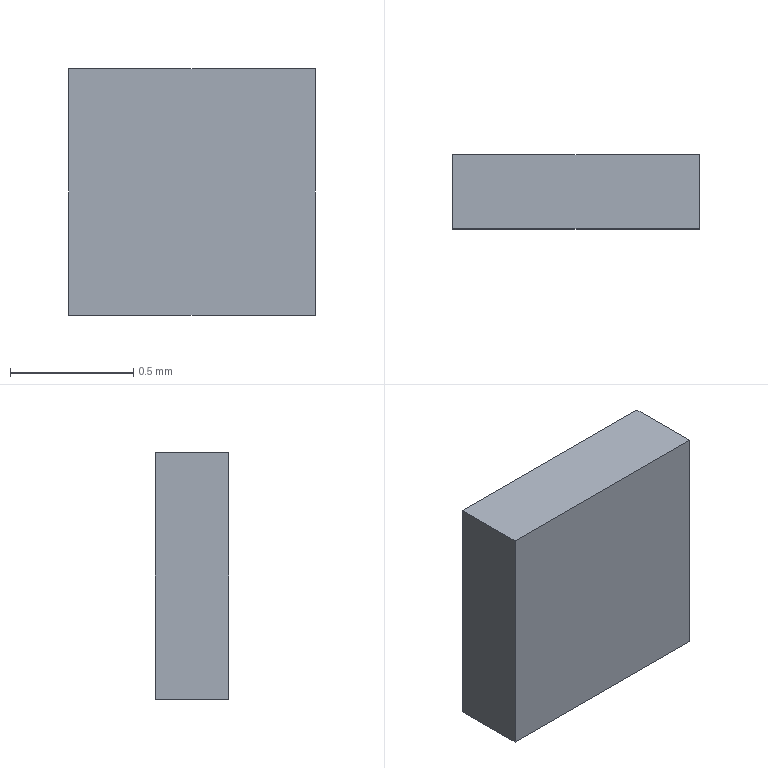Component | NX | SENSOR_21 | 1 solid | 6 faces | box 1 x 0.3 x 1 mm | volume 0 mm3 | plane 6
STEP:
#1=CARTESIAN_POINT('',(0.,0.,0.));
#2=DIRECTION('',(0.,0.,1.));
#3=DIRECTION('',(1.,0.,0.));
#4=AXIS2_PLACEMENT_3D('',#1,#2,#3);
#5=CARTESIAN_POINT('',(-590.087,100.903,1.));
#6=VERTEX_POINT('',#5);
#7=CARTESIAN_POINT('',(-591.087,100.903,1.));
#8=VERTEX_POINT('',#7);
#9=CARTESIAN_POINT('',(-590.587,100.903,1.));
#10=DIRECTION('',(-1.,0.,0.));
#11=VECTOR('',#10,1.);
#12=LINE('',#9,#11);
#13=CARTESIAN_POINT('',(-590.587,101.053,1.));
#14=DIRECTION('',(0.,0.,1.));
#15=DIRECTION('',(1.,0.,0.));
#16=AXIS2_PLACEMENT_3D('',#13,#14,#15);
#17=PLANE('',#16);
#18=CARTESIAN_POINT('',(0.,-0.15));
#19=DIRECTION('',(-1.,0.));
#20=VECTOR('',#19,1.);
#21=LINE('',#18,#20);
#22=(GEOMETRIC_REPRESENTATION_CONTEXT(2)PARAMETRIC_REPRESENTATION_CONTEXT()REPRESENTATION_CONTEXT('',''));
#23=DEFINITIONAL_REPRESENTATION('',(#21),#22);
#24=PCURVE('',#17,#23);
#25=CARTESIAN_POINT('',(-590.587,100.903,0.));
#26=DIRECTION('',(0.,-1.,0.));
#27=DIRECTION('',(0.,0.,-1.));
#28=AXIS2_PLACEMENT_3D('',#25,#26,#27);
#29=PLANE('',#28);
#30=CARTESIAN_POINT('',(-1.,0.));
#31=DIRECTION('',(0.,-1.));
#32=VECTOR('',#31,1.);
#33=LINE('',#30,#32);
#34=(GEOMETRIC_REPRESENTATION_CONTEXT(2)PARAMETRIC_REPRESENTATION_CONTEXT()REPRESENTATION_CONTEXT('',''));
#35=DEFINITIONAL_REPRESENTATION('',(#33),#34);
#36=PCURVE('',#29,#35);
#37=SURFACE_CURVE('',#12,(#24,#36),.PCURVE_S1.);
#38=EDGE_CURVE('',#6,#8,#37,.T.);
#39=ORIENTED_EDGE('',*,*,#38,.F.);
#40=CARTESIAN_POINT('',(-590.087,101.203,1.));
#41=VERTEX_POINT('',#40);
#42=CARTESIAN_POINT('',(-590.087,101.053,1.));
#43=DIRECTION('',(0.,-1.,0.));
#44=VECTOR('',#43,1.);
#45=LINE('',#42,#44);
#46=CARTESIAN_POINT('',(0.5,0.));
#47=DIRECTION('',(0.,-1.));
#48=VECTOR('',#47,1.);
#49=LINE('',#46,#48);
#50=(GEOMETRIC_REPRESENTATION_CONTEXT(2)PARAMETRIC_REPRESENTATION_CONTEXT()REPRESENTATION_CONTEXT('',''));
#51=DEFINITIONAL_REPRESENTATION('',(#49),#50);
#52=PCURVE('',#17,#51);
#53=CARTESIAN_POINT('',(-590.087,101.053,0.));
#54=DIRECTION('',(1.,0.,0.));
#55=DIRECTION('',(0.,0.,-1.));
#56=AXIS2_PLACEMENT_3D('',#53,#54,#55);
#57=PLANE('',#56);
#58=CARTESIAN_POINT('',(-1.,0.));
#59=DIRECTION('',(0.,-1.));
#60=VECTOR('',#59,1.);
#61=LINE('',#58,#60);
#62=(GEOMETRIC_REPRESENTATION_CONTEXT(2)PARAMETRIC_REPRESENTATION_CONTEXT()REPRESENTATION_CONTEXT('',''));
#63=DEFINITIONAL_REPRESENTATION('',(#61),#62);
#64=PCURVE('',#57,#63);
#65=SURFACE_CURVE('',#45,(#52,#64),.PCURVE_S1.);
#66=EDGE_CURVE('',#41,#6,#65,.T.);
#67=ORIENTED_EDGE('',*,*,#66,.F.);
#68=CARTESIAN_POINT('',(-591.087,101.203,1.));
#69=VERTEX_POINT('',#68);
#70=CARTESIAN_POINT('',(-590.587,101.203,1.));
#71=DIRECTION('',(1.,0.,0.));
#72=VECTOR('',#71,1.);
#73=LINE('',#70,#72);
#74=CARTESIAN_POINT('',(0.,0.15));
#75=DIRECTION('',(1.,0.));
#76=VECTOR('',#75,1.);
#77=LINE('',#74,#76);
#78=(GEOMETRIC_REPRESENTATION_CONTEXT(2)PARAMETRIC_REPRESENTATION_CONTEXT()REPRESENTATION_CONTEXT('',''));
#79=DEFINITIONAL_REPRESENTATION('',(#77),#78);
#80=PCURVE('',#17,#79);
#81=CARTESIAN_POINT('',(-590.587,101.203,0.));
#82=DIRECTION('',(0.,1.,0.));
#83=DIRECTION('',(0.,0.,1.));
#84=AXIS2_PLACEMENT_3D('',#81,#82,#83);
#85=PLANE('',#84);
#86=CARTESIAN_POINT('',(1.,0.));
#87=DIRECTION('',(0.,1.));
#88=VECTOR('',#87,1.);
#89=LINE('',#86,#88);
#90=(GEOMETRIC_REPRESENTATION_CONTEXT(2)PARAMETRIC_REPRESENTATION_CONTEXT()REPRESENTATION_CONTEXT('',''));
#91=DEFINITIONAL_REPRESENTATION('',(#89),#90);
#92=PCURVE('',#85,#91);
#93=SURFACE_CURVE('',#73,(#80,#92),.PCURVE_S1.);
#94=EDGE_CURVE('',#69,#41,#93,.T.);
#95=ORIENTED_EDGE('',*,*,#94,.F.);
#96=CARTESIAN_POINT('',(-591.087,101.053,1.));
#97=DIRECTION('',(0.,1.,0.));
#98=VECTOR('',#97,1.);
#99=LINE('',#96,#98);
#100=CARTESIAN_POINT('',(-0.5,0.));
#101=DIRECTION('',(0.,1.));
#102=VECTOR('',#101,1.);
#103=LINE('',#100,#102);
#104=(GEOMETRIC_REPRESENTATION_CONTEXT(2)PARAMETRIC_REPRESENTATION_CONTEXT()REPRESENTATION_CONTEXT('',''));
#105=DEFINITIONAL_REPRESENTATION('',(#103),#104);
#106=PCURVE('',#17,#105);
#107=CARTESIAN_POINT('',(-591.087,101.053,0.));
#108=DIRECTION('',(-1.,0.,0.));
#109=DIRECTION('',(0.,0.,1.));
#110=AXIS2_PLACEMENT_3D('',#107,#108,#109);
#111=PLANE('',#110);
#112=CARTESIAN_POINT('',(1.,0.));
#113=DIRECTION('',(0.,1.));
#114=VECTOR('',#113,1.);
#115=LINE('',#112,#114);
#116=(GEOMETRIC_REPRESENTATION_CONTEXT(2)PARAMETRIC_REPRESENTATION_CONTEXT()REPRESENTATION_CONTEXT('',''));
#117=DEFINITIONAL_REPRESENTATION('',(#115),#116);
#118=PCURVE('',#111,#117);
#119=SURFACE_CURVE('',#99,(#106,#118),.PCURVE_S1.);
#120=EDGE_CURVE('',#8,#69,#119,.T.);
#121=ORIENTED_EDGE('',*,*,#120,.F.);
#122=EDGE_LOOP('',(#39,#67,#95,#121));
#123=FACE_BOUND('',#122,.T.);
#124=ADVANCED_FACE('',(#123),#17,.T.);
#125=CARTESIAN_POINT('',(-590.087,100.903,0.));
#126=VERTEX_POINT('',#125);
#127=CARTESIAN_POINT('',(-590.087,100.903,0.));
#128=DIRECTION('',(0.,0.,1.));
#129=VECTOR('',#128,1.);
#130=LINE('',#127,#129);
#131=CARTESIAN_POINT('',(0.,0.5));
#132=DIRECTION('',(-1.,0.));
#133=VECTOR('',#132,1.);
#134=LINE('',#131,#133);
#135=(GEOMETRIC_REPRESENTATION_CONTEXT(2)PARAMETRIC_REPRESENTATION_CONTEXT()REPRESENTATION_CONTEXT('',''));
#136=DEFINITIONAL_REPRESENTATION('',(#134),#135);
#137=PCURVE('',#29,#136);
#138=CARTESIAN_POINT('',(0.,-0.15));
#139=DIRECTION('',(-1.,0.));
#140=VECTOR('',#139,1.);
#141=LINE('',#138,#140);
#142=(GEOMETRIC_REPRESENTATION_CONTEXT(2)PARAMETRIC_REPRESENTATION_CONTEXT()REPRESENTATION_CONTEXT('',''));
#143=DEFINITIONAL_REPRESENTATION('',(#141),#142);
#144=PCURVE('',#57,#143);
#145=SURFACE_CURVE('',#130,(#137,#144),.PCURVE_S1.);
#146=EDGE_CURVE('',#126,#6,#145,.T.);
#147=ORIENTED_EDGE('',*,*,#146,.T.);
#148=ORIENTED_EDGE('',*,*,#38,.T.);
#149=CARTESIAN_POINT('',(-591.087,100.903,0.));
#150=VERTEX_POINT('',#149);
#151=CARTESIAN_POINT('',(-591.087,100.903,0.));
#152=DIRECTION('',(0.,0.,1.));
#153=VECTOR('',#152,1.);
#154=LINE('',#151,#153);
#155=CARTESIAN_POINT('',(0.,-0.5));
#156=DIRECTION('',(-1.,0.));
#157=VECTOR('',#156,1.);
#158=LINE('',#155,#157);
#159=(GEOMETRIC_REPRESENTATION_CONTEXT(2)PARAMETRIC_REPRESENTATION_CONTEXT()REPRESENTATION_CONTEXT('',''));
#160=DEFINITIONAL_REPRESENTATION('',(#158),#159);
#161=PCURVE('',#29,#160);
#162=CARTESIAN_POINT('',(0.,-0.15));
#163=DIRECTION('',(1.,0.));
#164=VECTOR('',#163,1.);
#165=LINE('',#162,#164);
#166=(GEOMETRIC_REPRESENTATION_CONTEXT(2)PARAMETRIC_REPRESENTATION_CONTEXT()REPRESENTATION_CONTEXT('',''));
#167=DEFINITIONAL_REPRESENTATION('',(#165),#166);
#168=PCURVE('',#111,#167);
#169=SURFACE_CURVE('',#154,(#161,#168),.PCURVE_S1.);
#170=EDGE_CURVE('',#150,#8,#169,.T.);
#171=ORIENTED_EDGE('',*,*,#170,.F.);
#172=CARTESIAN_POINT('',(-590.587,100.903,0.));
#173=DIRECTION('',(1.,0.,0.));
#174=VECTOR('',#173,1.);
#175=LINE('',#172,#174);
#176=CARTESIAN_POINT('',(0.,0.));
#177=DIRECTION('',(0.,1.));
#178=VECTOR('',#177,1.);
#179=LINE('',#176,#178);
#180=(GEOMETRIC_REPRESENTATION_CONTEXT(2)PARAMETRIC_REPRESENTATION_CONTEXT()REPRESENTATION_CONTEXT('',''));
#181=DEFINITIONAL_REPRESENTATION('',(#179),#180);
#182=PCURVE('',#29,#181);
#183=CARTESIAN_POINT('',(-590.587,101.053,0.));
#184=DIRECTION('',(0.,0.,-1.));
#185=DIRECTION('',(-1.,0.,0.));
#186=AXIS2_PLACEMENT_3D('',#183,#184,#185);
#187=PLANE('',#186);
#188=CARTESIAN_POINT('',(0.,-0.15));
#189=DIRECTION('',(-1.,0.));
#190=VECTOR('',#189,1.);
#191=LINE('',#188,#190);
#192=(GEOMETRIC_REPRESENTATION_CONTEXT(2)PARAMETRIC_REPRESENTATION_CONTEXT()REPRESENTATION_CONTEXT('',''));
#193=DEFINITIONAL_REPRESENTATION('',(#191),#192);
#194=PCURVE('',#187,#193);
#195=SURFACE_CURVE('',#175,(#182,#194),.PCURVE_S1.);
#196=EDGE_CURVE('',#150,#126,#195,.T.);
#197=ORIENTED_EDGE('',*,*,#196,.T.);
#198=EDGE_LOOP('',(#147,#148,#171,#197));
#199=FACE_BOUND('',#198,.T.);
#200=ADVANCED_FACE('',(#199),#29,.T.);
#201=ORIENTED_EDGE('',*,*,#170,.T.);
#202=ORIENTED_EDGE('',*,*,#120,.T.);
#203=CARTESIAN_POINT('',(-591.087,101.203,0.));
#204=VERTEX_POINT('',#203);
#205=CARTESIAN_POINT('',(-591.087,101.203,0.));
#206=DIRECTION('',(0.,0.,1.));
#207=VECTOR('',#206,1.);
#208=LINE('',#205,#207);
#209=CARTESIAN_POINT('',(0.,0.15));
#210=DIRECTION('',(1.,0.));
#211=VECTOR('',#210,1.);
#212=LINE('',#209,#211);
#213=(GEOMETRIC_REPRESENTATION_CONTEXT(2)PARAMETRIC_REPRESENTATION_CONTEXT()REPRESENTATION_CONTEXT('',''));
#214=DEFINITIONAL_REPRESENTATION('',(#212),#213);
#215=PCURVE('',#111,#214);
#216=CARTESIAN_POINT('',(0.,-0.5));
#217=DIRECTION('',(1.,0.));
#218=VECTOR('',#217,1.);
#219=LINE('',#216,#218);
#220=(GEOMETRIC_REPRESENTATION_CONTEXT(2)PARAMETRIC_REPRESENTATION_CONTEXT()REPRESENTATION_CONTEXT('',''));
#221=DEFINITIONAL_REPRESENTATION('',(#219),#220);
#222=PCURVE('',#85,#221);
#223=SURFACE_CURVE('',#208,(#215,#222),.PCURVE_S1.);
#224=EDGE_CURVE('',#204,#69,#223,.T.);
#225=ORIENTED_EDGE('',*,*,#224,.F.);
#226=CARTESIAN_POINT('',(-591.087,101.053,0.));
#227=DIRECTION('',(0.,-1.,0.));
#228=VECTOR('',#227,1.);
#229=LINE('',#226,#228);
#230=CARTESIAN_POINT('',(0.,0.));
#231=DIRECTION('',(0.,-1.));
#232=VECTOR('',#231,1.);
#233=LINE('',#230,#232);
#234=(GEOMETRIC_REPRESENTATION_CONTEXT(2)PARAMETRIC_REPRESENTATION_CONTEXT()REPRESENTATION_CONTEXT('',''));
#235=DEFINITIONAL_REPRESENTATION('',(#233),#234);
#236=PCURVE('',#111,#235);
#237=CARTESIAN_POINT('',(0.5,0.));
#238=DIRECTION('',(0.,-1.));
#239=VECTOR('',#238,1.);
#240=LINE('',#237,#239);
#241=(GEOMETRIC_REPRESENTATION_CONTEXT(2)PARAMETRIC_REPRESENTATION_CONTEXT()REPRESENTATION_CONTEXT('',''));
#242=DEFINITIONAL_REPRESENTATION('',(#240),#241);
#243=PCURVE('',#187,#242);
#244=SURFACE_CURVE('',#229,(#236,#243),.PCURVE_S1.);
#245=EDGE_CURVE('',#204,#150,#244,.T.);
#246=ORIENTED_EDGE('',*,*,#245,.T.);
#247=EDGE_LOOP('',(#201,#202,#225,#246));
#248=FACE_BOUND('',#247,.T.);
#249=ADVANCED_FACE('',(#248),#111,.T.);
#250=ORIENTED_EDGE('',*,*,#224,.T.);
#251=ORIENTED_EDGE('',*,*,#94,.T.);
#252=CARTESIAN_POINT('',(-590.087,101.203,0.));
#253=VERTEX_POINT('',#252);
#254=CARTESIAN_POINT('',(-590.087,101.203,0.));
#255=DIRECTION('',(0.,0.,1.));
#256=VECTOR('',#255,1.);
#257=LINE('',#254,#256);
#258=CARTESIAN_POINT('',(0.,0.5));
#259=DIRECTION('',(1.,0.));
#260=VECTOR('',#259,1.);
#261=LINE('',#258,#260);
#262=(GEOMETRIC_REPRESENTATION_CONTEXT(2)PARAMETRIC_REPRESENTATION_CONTEXT()REPRESENTATION_CONTEXT('',''));
#263=DEFINITIONAL_REPRESENTATION('',(#261),#262);
#264=PCURVE('',#85,#263);
#265=CARTESIAN_POINT('',(0.,0.15));
#266=DIRECTION('',(-1.,0.));
#267=VECTOR('',#266,1.);
#268=LINE('',#265,#267);
#269=(GEOMETRIC_REPRESENTATION_CONTEXT(2)PARAMETRIC_REPRESENTATION_CONTEXT()REPRESENTATION_CONTEXT('',''));
#270=DEFINITIONAL_REPRESENTATION('',(#268),#269);
#271=PCURVE('',#57,#270);
#272=SURFACE_CURVE('',#257,(#264,#271),.PCURVE_S1.);
#273=EDGE_CURVE('',#253,#41,#272,.T.);
#274=ORIENTED_EDGE('',*,*,#273,.F.);
#275=CARTESIAN_POINT('',(-590.587,101.203,0.));
#276=DIRECTION('',(-1.,0.,0.));
#277=VECTOR('',#276,1.);
#278=LINE('',#275,#277);
#279=CARTESIAN_POINT('',(0.,0.));
#280=DIRECTION('',(0.,-1.));
#281=VECTOR('',#280,1.);
#282=LINE('',#279,#281);
#283=(GEOMETRIC_REPRESENTATION_CONTEXT(2)PARAMETRIC_REPRESENTATION_CONTEXT()REPRESENTATION_CONTEXT('',''));
#284=DEFINITIONAL_REPRESENTATION('',(#282),#283);
#285=PCURVE('',#85,#284);
#286=CARTESIAN_POINT('',(0.,0.15));
#287=DIRECTION('',(1.,0.));
#288=VECTOR('',#287,1.);
#289=LINE('',#286,#288);
#290=(GEOMETRIC_REPRESENTATION_CONTEXT(2)PARAMETRIC_REPRESENTATION_CONTEXT()REPRESENTATION_CONTEXT('',''));
#291=DEFINITIONAL_REPRESENTATION('',(#289),#290);
#292=PCURVE('',#187,#291);
#293=SURFACE_CURVE('',#278,(#285,#292),.PCURVE_S1.);
#294=EDGE_CURVE('',#253,#204,#293,.T.);
#295=ORIENTED_EDGE('',*,*,#294,.T.);
#296=EDGE_LOOP('',(#250,#251,#274,#295));
#297=FACE_BOUND('',#296,.T.);
#298=ADVANCED_FACE('',(#297),#85,.T.);
#299=CARTESIAN_POINT('',(-590.087,101.053,0.));
#300=DIRECTION('',(0.,1.,0.));
#301=VECTOR('',#300,1.);
#302=LINE('',#299,#301);
#303=CARTESIAN_POINT('',(-0.5,0.));
#304=DIRECTION('',(0.,1.));
#305=VECTOR('',#304,1.);
#306=LINE('',#303,#305);
#307=(GEOMETRIC_REPRESENTATION_CONTEXT(2)PARAMETRIC_REPRESENTATION_CONTEXT()REPRESENTATION_CONTEXT('',''));
#308=DEFINITIONAL_REPRESENTATION('',(#306),#307);
#309=PCURVE('',#187,#308);
#310=CARTESIAN_POINT('',(0.,0.));
#311=DIRECTION('',(0.,1.));
#312=VECTOR('',#311,1.);
#313=LINE('',#310,#312);
#314=(GEOMETRIC_REPRESENTATION_CONTEXT(2)PARAMETRIC_REPRESENTATION_CONTEXT()REPRESENTATION_CONTEXT('',''));
#315=DEFINITIONAL_REPRESENTATION('',(#313),#314);
#316=PCURVE('',#57,#315);
#317=SURFACE_CURVE('',#302,(#309,#316),.PCURVE_S1.);
#318=EDGE_CURVE('',#126,#253,#317,.T.);
#319=ORIENTED_EDGE('',*,*,#318,.F.);
#320=ORIENTED_EDGE('',*,*,#196,.F.);
#321=ORIENTED_EDGE('',*,*,#245,.F.);
#322=ORIENTED_EDGE('',*,*,#294,.F.);
#323=EDGE_LOOP('',(#319,#320,#321,#322));
#324=FACE_BOUND('',#323,.T.);
#325=ADVANCED_FACE('',(#324),#187,.T.);
#326=ORIENTED_EDGE('',*,*,#318,.T.);
#327=ORIENTED_EDGE('',*,*,#273,.T.);
#328=ORIENTED_EDGE('',*,*,#66,.T.);
#329=ORIENTED_EDGE('',*,*,#146,.F.);
#330=EDGE_LOOP('',(#326,#327,#328,#329));
#331=FACE_BOUND('',#330,.T.);
#332=ADVANCED_FACE('',(#331),#57,.T.);
#333=CLOSED_SHELL('',(#124,#200,#249,#298,#325,#332));
#334=MANIFOLD_SOLID_BREP('',#333);
#335=(LENGTH_UNIT()NAMED_UNIT(*)SI_UNIT(.MILLI.,.METRE.));
#336=UNCERTAINTY_MEASURE_WITH_UNIT(LENGTH_MEASURE(0.0000001),#335,'','');
#337=(NAMED_UNIT(*)PLANE_ANGLE_UNIT()SI_UNIT($,.RADIAN.));
#338=(NAMED_UNIT(*)SI_UNIT($,.STERADIAN.)SOLID_ANGLE_UNIT());
#339=(GEOMETRIC_REPRESENTATION_CONTEXT(3)GLOBAL_UNCERTAINTY_ASSIGNED_CONTEXT((#336))GLOBAL_UNIT_ASSIGNED_CONTEXT((#335,#337,#338))REPRESENTATION_CONTEXT('',''));
#340=ADVANCED_BREP_SHAPE_REPRESENTATION('',(#4,#334),#339);